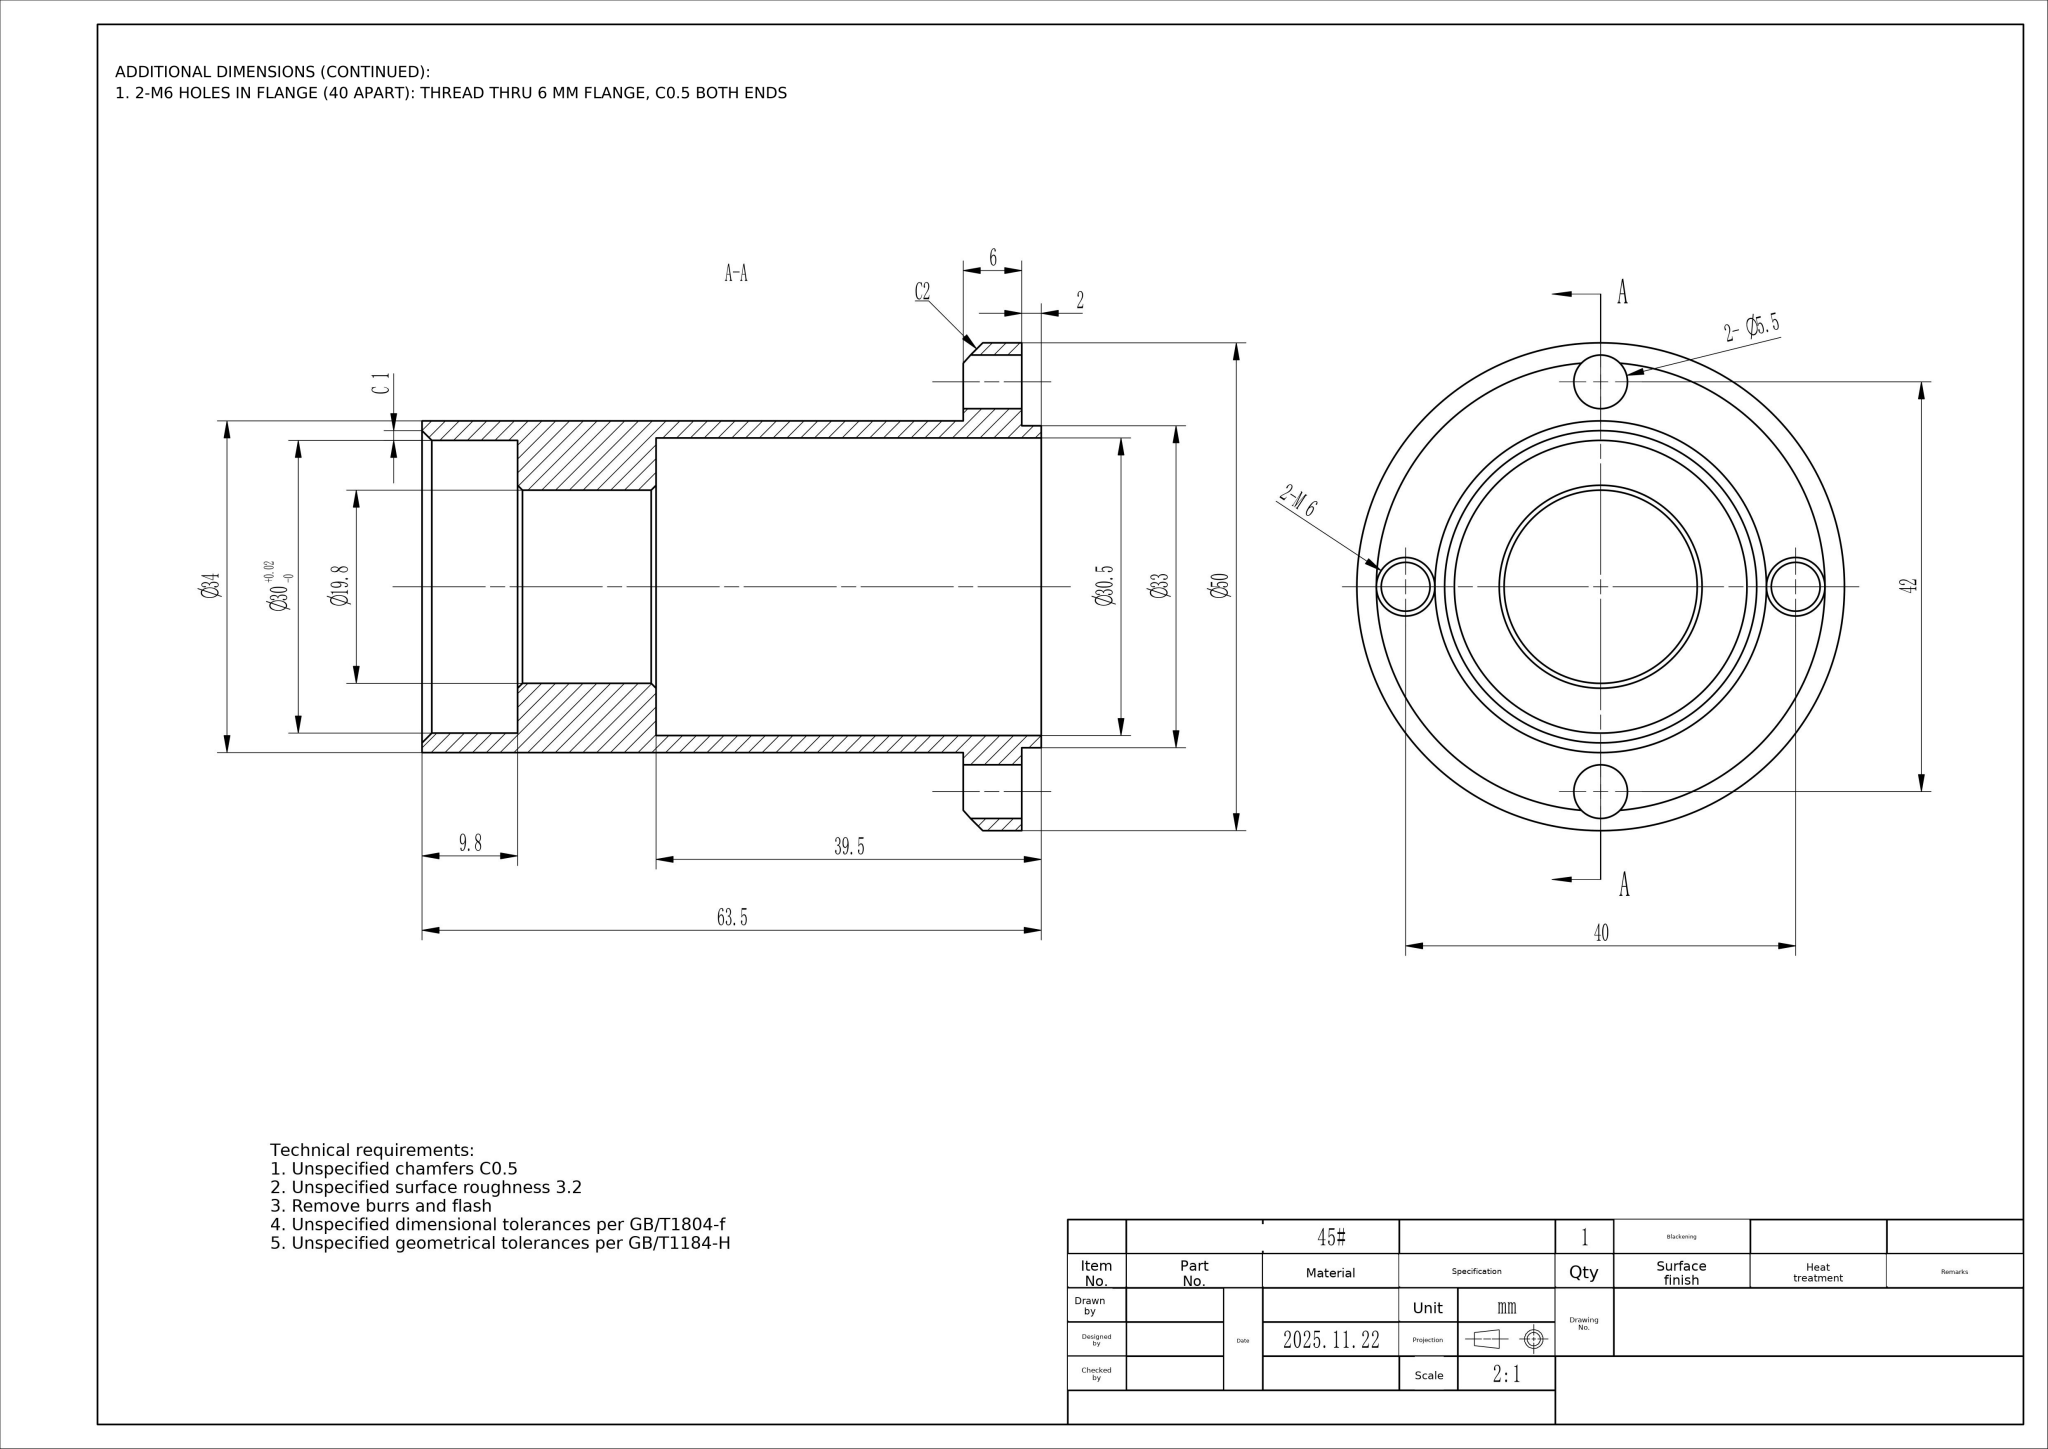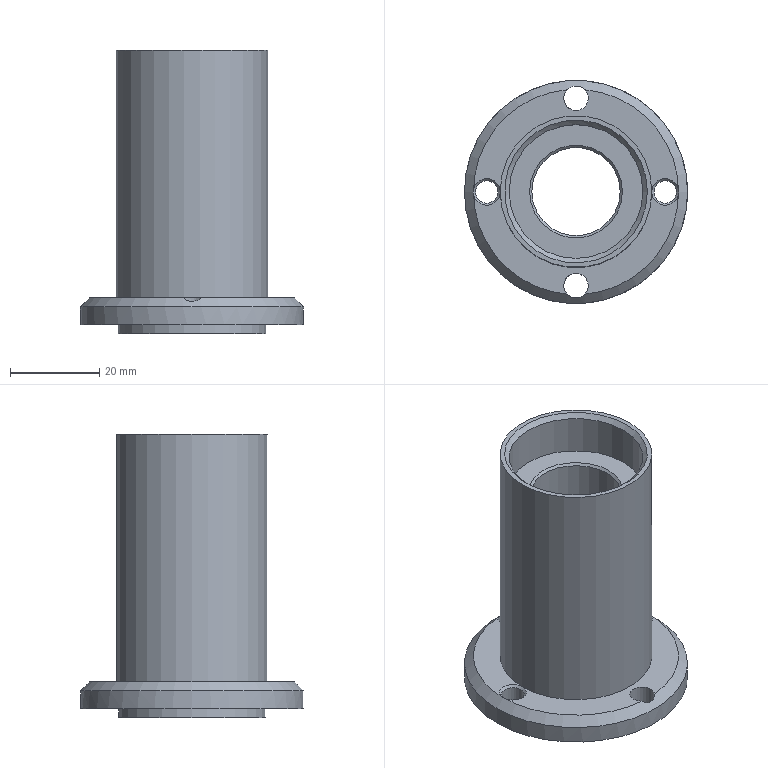Part | NX | mm | 1 solid | 25 faces | box 50 x 50 x 63.5 mm | volume 22825 mm3 | cylinder 10 | cone 8 | plane 7 | commonest cylinder face diameters 5.5 x2 5 x2 19.8 x1 30.5 x1 33 x1 50 x1 34 x1 30 x1
STEP:
#1=CARTESIAN_POINT('',(0.,0.,0.));
#2=DIRECTION('',(0.,0.,1.));
#3=DIRECTION('',(1.,0.,0.));
#4=AXIS2_PLACEMENT_3D('',#1,#2,#3);
#5=(LENGTH_UNIT()NAMED_UNIT(*)SI_UNIT(.MILLI.,.METRE.));
#6=UNCERTAINTY_MEASURE_WITH_UNIT(LENGTH_MEASURE(0.0508),#5,'','');
#7=(NAMED_UNIT(*)PLANE_ANGLE_UNIT()SI_UNIT($,.RADIAN.));
#8=PLANE_ANGLE_MEASURE_WITH_UNIT(PLANE_ANGLE_MEASURE(0.01745),#7);
#9=DIMENSIONAL_EXPONENTS(0.,0.,0.,0.,0.,0.,0.);
#10=(CONVERSION_BASED_UNIT('',#8)NAMED_UNIT(#9)PLANE_ANGLE_UNIT());
#11=(NAMED_UNIT(*)SI_UNIT($,.STERADIAN.)SOLID_ANGLE_UNIT());
#12=(GEOMETRIC_REPRESENTATION_CONTEXT(3)GLOBAL_UNCERTAINTY_ASSIGNED_CONTEXT((#6))GLOBAL_UNIT_ASSIGNED_CONTEXT((#5,#10,#11))REPRESENTATION_CONTEXT('',''));
#13=SHAPE_REPRESENTATION('',(#4),#12);
#14=CARTESIAN_POINT('',(-1.973,22.915,-55.5));
#15=VERTEX_POINT('',#14);
#16=CARTESIAN_POINT('',(1.973,22.915,-55.5));
#17=VERTEX_POINT('',#16);
#18=CARTESIAN_POINT('',(0.,21.,-55.5));
#19=DIRECTION('',(0.,0.,1.));
#20=DIRECTION('',(1.,0.,0.));
#21=AXIS2_PLACEMENT_3D('',#18,#19,#20);
#22=CIRCLE('',#21,2.75);
#23=EDGE_CURVE('',#15,#17,#22,.T.);
#24=ORIENTED_EDGE('',*,*,#23,.F.);
#25=CARTESIAN_POINT('',(-23.,0.,-55.5));
#26=VERTEX_POINT('',#25);
#27=CARTESIAN_POINT('',(0.,0.,-55.5));
#28=DIRECTION('',(0.,0.,1.));
#29=DIRECTION('',(1.,0.,0.));
#30=AXIS2_PLACEMENT_3D('',#27,#28,#29);
#31=CIRCLE('',#30,23.);
#32=EDGE_CURVE('',#15,#26,#31,.T.);
#33=ORIENTED_EDGE('',*,*,#32,.T.);
#34=CARTESIAN_POINT('',(-17.,0.,-55.5));
#35=VERTEX_POINT('',#34);
#36=CARTESIAN_POINT('',(-20.,0.,-55.5));
#37=DIRECTION('',(0.,0.,-1.));
#38=DIRECTION('',(1.,0.,0.));
#39=AXIS2_PLACEMENT_3D('',#36,#37,#38);
#40=CIRCLE('',#39,3.);
#41=EDGE_CURVE('',#26,#35,#40,.T.);
#42=ORIENTED_EDGE('',*,*,#41,.T.);
#43=CARTESIAN_POINT('',(17.,0.,-55.5));
#44=VERTEX_POINT('',#43);
#45=CARTESIAN_POINT('',(0.,0.,-55.5));
#46=DIRECTION('',(0.,0.,1.));
#47=DIRECTION('',(-1.,0.,0.));
#48=AXIS2_PLACEMENT_3D('',#45,#46,#47);
#49=CIRCLE('',#48,17.);
#50=EDGE_CURVE('',#44,#35,#49,.T.);
#51=ORIENTED_EDGE('',*,*,#50,.F.);
#52=CARTESIAN_POINT('',(23.,0.,-55.5));
#53=VERTEX_POINT('',#52);
#54=CARTESIAN_POINT('',(20.,0.,-55.5));
#55=DIRECTION('',(0.,0.,-1.));
#56=DIRECTION('',(1.,0.,0.));
#57=AXIS2_PLACEMENT_3D('',#54,#55,#56);
#58=CIRCLE('',#57,3.);
#59=EDGE_CURVE('',#44,#53,#58,.T.);
#60=ORIENTED_EDGE('',*,*,#59,.T.);
#61=CARTESIAN_POINT('',(0.,0.,-55.5));
#62=DIRECTION('',(0.,0.,1.));
#63=DIRECTION('',(1.,0.,0.));
#64=AXIS2_PLACEMENT_3D('',#61,#62,#63);
#65=CIRCLE('',#64,23.);
#66=EDGE_CURVE('',#53,#17,#65,.T.);
#67=ORIENTED_EDGE('',*,*,#66,.T.);
#68=EDGE_LOOP('',(#24,#33,#42,#51,#60,#67));
#69=FACE_OUTER_BOUND('',#68,.T.);
#70=CARTESIAN_POINT('',(0.,25.,-55.5));
#71=DIRECTION('',(0.,0.,1.));
#72=DIRECTION('',(1.,0.,0.));
#73=AXIS2_PLACEMENT_3D('',#70,#71,#72);
#74=PLANE('',#73);
#75=ADVANCED_FACE('',(#69),#74,.T.);
#76=CARTESIAN_POINT('',(-9.9,0.,-23.5));
#77=VERTEX_POINT('',#76);
#78=CARTESIAN_POINT('',(0.,0.,-23.5));
#79=DIRECTION('',(0.,0.,-1.));
#80=DIRECTION('',(-1.,0.,0.));
#81=AXIS2_PLACEMENT_3D('',#78,#79,#80);
#82=CIRCLE('',#81,9.9);
#83=EDGE_CURVE('',#77,#77,#82,.T.);
#84=ORIENTED_EDGE('',*,*,#83,.T.);
#85=EDGE_LOOP('',(#84));
#86=FACE_BOUND('',#85,.T.);
#87=CARTESIAN_POINT('',(9.9,0.,-10.3));
#88=VERTEX_POINT('',#87);
#89=CARTESIAN_POINT('',(0.,0.,-10.3));
#90=DIRECTION('',(0.,0.,1.));
#91=DIRECTION('',(1.,0.,0.));
#92=AXIS2_PLACEMENT_3D('',#89,#90,#91);
#93=CIRCLE('',#92,9.9);
#94=EDGE_CURVE('',#88,#88,#93,.T.);
#95=ORIENTED_EDGE('',*,*,#94,.T.);
#96=EDGE_LOOP('',(#95));
#97=FACE_BOUND('',#96,.T.);
#98=CARTESIAN_POINT('',(0.,0.,0.));
#99=DIRECTION('',(0.,0.,-1.));
#100=DIRECTION('',(-1.,0.,0.));
#101=AXIS2_PLACEMENT_3D('',#98,#99,#100);
#102=CYLINDRICAL_SURFACE('',#101,9.9);
#103=ADVANCED_FACE('',(#86,#97),#102,.F.);
#104=CARTESIAN_POINT('',(-10.4,0.,-24.));
#105=VERTEX_POINT('',#104);
#106=CARTESIAN_POINT('',(0.,0.,-24.));
#107=DIRECTION('',(0.,0.,1.));
#108=DIRECTION('',(-1.,0.,0.));
#109=AXIS2_PLACEMENT_3D('',#106,#107,#108);
#110=CIRCLE('',#109,10.4);
#111=EDGE_CURVE('',#105,#105,#110,.T.);
#112=ORIENTED_EDGE('',*,*,#111,.T.);
#113=EDGE_LOOP('',(#112));
#114=FACE_BOUND('',#113,.T.);
#115=CARTESIAN_POINT('',(-15.25,0.,-24.));
#116=VERTEX_POINT('',#115);
#117=CARTESIAN_POINT('',(0.,0.,-24.));
#118=DIRECTION('',(0.,0.,1.));
#119=DIRECTION('',(-1.,0.,0.));
#120=AXIS2_PLACEMENT_3D('',#117,#118,#119);
#121=CIRCLE('',#120,15.25);
#122=EDGE_CURVE('',#116,#116,#121,.T.);
#123=ORIENTED_EDGE('',*,*,#122,.F.);
#124=EDGE_LOOP('',(#123));
#125=FACE_BOUND('',#124,.T.);
#126=CARTESIAN_POINT('',(0.,9.9,-24.));
#127=DIRECTION('',(0.,0.,-1.));
#128=DIRECTION('',(-1.,0.,0.));
#129=AXIS2_PLACEMENT_3D('',#126,#127,#128);
#130=PLANE('',#129);
#131=ADVANCED_FACE('',(#114,#125),#130,.T.);
#132=CARTESIAN_POINT('',(-15.25,0.,-63.5));
#133=VERTEX_POINT('',#132);
#134=CARTESIAN_POINT('',(0.,0.,-63.5));
#135=DIRECTION('',(0.,0.,1.));
#136=DIRECTION('',(-1.,0.,0.));
#137=AXIS2_PLACEMENT_3D('',#134,#135,#136);
#138=CIRCLE('',#137,15.25);
#139=EDGE_CURVE('',#133,#133,#138,.T.);
#140=ORIENTED_EDGE('',*,*,#139,.F.);
#141=EDGE_LOOP('',(#140));
#142=FACE_BOUND('',#141,.T.);
#143=ORIENTED_EDGE('',*,*,#122,.T.);
#144=EDGE_LOOP('',(#143));
#145=FACE_BOUND('',#144,.T.);
#146=CARTESIAN_POINT('',(0.,0.,0.));
#147=DIRECTION('',(0.,0.,-1.));
#148=DIRECTION('',(-1.,0.,0.));
#149=AXIS2_PLACEMENT_3D('',#146,#147,#148);
#150=CYLINDRICAL_SURFACE('',#149,15.25);
#151=ADVANCED_FACE('',(#142,#145),#150,.F.);
#152=CARTESIAN_POINT('',(-16.5,0.,-63.5));
#153=VERTEX_POINT('',#152);
#154=CARTESIAN_POINT('',(0.,0.,-63.5));
#155=DIRECTION('',(0.,0.,1.));
#156=DIRECTION('',(-1.,0.,0.));
#157=AXIS2_PLACEMENT_3D('',#154,#155,#156);
#158=CIRCLE('',#157,16.5);
#159=EDGE_CURVE('',#153,#153,#158,.T.);
#160=ORIENTED_EDGE('',*,*,#159,.F.);
#161=EDGE_LOOP('',(#160));
#162=FACE_BOUND('',#161,.T.);
#163=ORIENTED_EDGE('',*,*,#139,.T.);
#164=EDGE_LOOP('',(#163));
#165=FACE_BOUND('',#164,.T.);
#166=CARTESIAN_POINT('',(0.,15.25,-63.5));
#167=DIRECTION('',(0.,0.,-1.));
#168=DIRECTION('',(-1.,0.,0.));
#169=AXIS2_PLACEMENT_3D('',#166,#167,#168);
#170=PLANE('',#169);
#171=ADVANCED_FACE('',(#162,#165),#170,.T.);
#172=CARTESIAN_POINT('',(-16.5,0.,-61.5));
#173=VERTEX_POINT('',#172);
#174=CARTESIAN_POINT('',(0.,0.,-61.5));
#175=DIRECTION('',(0.,0.,1.));
#176=DIRECTION('',(-1.,0.,0.));
#177=AXIS2_PLACEMENT_3D('',#174,#175,#176);
#178=CIRCLE('',#177,16.5);
#179=EDGE_CURVE('',#173,#173,#178,.T.);
#180=ORIENTED_EDGE('',*,*,#179,.F.);
#181=EDGE_LOOP('',(#180));
#182=FACE_BOUND('',#181,.T.);
#183=ORIENTED_EDGE('',*,*,#159,.T.);
#184=EDGE_LOOP('',(#183));
#185=FACE_BOUND('',#184,.T.);
#186=CARTESIAN_POINT('',(0.,0.,0.));
#187=DIRECTION('',(0.,0.,-1.));
#188=DIRECTION('',(-1.,0.,0.));
#189=AXIS2_PLACEMENT_3D('',#186,#187,#188);
#190=CYLINDRICAL_SURFACE('',#189,16.5);
#191=ADVANCED_FACE('',(#182,#185),#190,.T.);
#192=CARTESIAN_POINT('',(17.,0.,-61.5));
#193=VERTEX_POINT('',#192);
#194=CARTESIAN_POINT('',(20.,0.,-61.5));
#195=DIRECTION('',(0.,0.,1.));
#196=DIRECTION('',(-1.,0.,0.));
#197=AXIS2_PLACEMENT_3D('',#194,#195,#196);
#198=CIRCLE('',#197,3.);
#199=EDGE_CURVE('',#193,#193,#198,.T.);
#200=ORIENTED_EDGE('',*,*,#199,.T.);
#201=EDGE_LOOP('',(#200));
#202=FACE_BOUND('',#201,.T.);
#203=CARTESIAN_POINT('',(-23.,0.,-61.5));
#204=VERTEX_POINT('',#203);
#205=CARTESIAN_POINT('',(-20.,0.,-61.5));
#206=DIRECTION('',(0.,0.,1.));
#207=DIRECTION('',(-1.,0.,0.));
#208=AXIS2_PLACEMENT_3D('',#205,#206,#207);
#209=CIRCLE('',#208,3.);
#210=EDGE_CURVE('',#204,#204,#209,.T.);
#211=ORIENTED_EDGE('',*,*,#210,.T.);
#212=EDGE_LOOP('',(#211));
#213=FACE_BOUND('',#212,.T.);
#214=CARTESIAN_POINT('',(-2.75,-21.,-61.5));
#215=VERTEX_POINT('',#214);
#216=CARTESIAN_POINT('',(0.,-21.,-61.5));
#217=DIRECTION('',(0.,0.,-1.));
#218=DIRECTION('',(-1.,0.,0.));
#219=AXIS2_PLACEMENT_3D('',#216,#217,#218);
#220=CIRCLE('',#219,2.75);
#221=EDGE_CURVE('',#215,#215,#220,.T.);
#222=ORIENTED_EDGE('',*,*,#221,.F.);
#223=EDGE_LOOP('',(#222));
#224=FACE_BOUND('',#223,.T.);
#225=CARTESIAN_POINT('',(-2.75,21.,-61.5));
#226=VERTEX_POINT('',#225);
#227=CARTESIAN_POINT('',(0.,21.,-61.5));
#228=DIRECTION('',(0.,0.,-1.));
#229=DIRECTION('',(-1.,0.,0.));
#230=AXIS2_PLACEMENT_3D('',#227,#228,#229);
#231=CIRCLE('',#230,2.75);
#232=EDGE_CURVE('',#226,#226,#231,.T.);
#233=ORIENTED_EDGE('',*,*,#232,.F.);
#234=EDGE_LOOP('',(#233));
#235=FACE_BOUND('',#234,.T.);
#236=CARTESIAN_POINT('',(-25.,0.,-61.5));
#237=VERTEX_POINT('',#236);
#238=CARTESIAN_POINT('',(0.,0.,-61.5));
#239=DIRECTION('',(0.,0.,1.));
#240=DIRECTION('',(-1.,0.,0.));
#241=AXIS2_PLACEMENT_3D('',#238,#239,#240);
#242=CIRCLE('',#241,25.);
#243=EDGE_CURVE('',#237,#237,#242,.T.);
#244=ORIENTED_EDGE('',*,*,#243,.F.);
#245=EDGE_LOOP('',(#244));
#246=FACE_BOUND('',#245,.T.);
#247=ORIENTED_EDGE('',*,*,#179,.T.);
#248=EDGE_LOOP('',(#247));
#249=FACE_BOUND('',#248,.T.);
#250=CARTESIAN_POINT('',(0.,16.5,-61.5));
#251=DIRECTION('',(0.,0.,-1.));
#252=DIRECTION('',(-1.,0.,0.));
#253=AXIS2_PLACEMENT_3D('',#250,#251,#252);
#254=PLANE('',#253);
#255=ADVANCED_FACE('',(#202,#213,#224,#235,#246,#249),#254,.T.);
#256=CARTESIAN_POINT('',(25.,0.,-57.5));
#257=VERTEX_POINT('',#256);
#258=CARTESIAN_POINT('',(0.,0.,-57.5));
#259=DIRECTION('',(0.,0.,-1.));
#260=DIRECTION('',(1.,0.,0.));
#261=AXIS2_PLACEMENT_3D('',#258,#259,#260);
#262=CIRCLE('',#261,25.);
#263=EDGE_CURVE('',#257,#257,#262,.T.);
#264=ORIENTED_EDGE('',*,*,#263,.T.);
#265=EDGE_LOOP('',(#264));
#266=FACE_BOUND('',#265,.T.);
#267=ORIENTED_EDGE('',*,*,#243,.T.);
#268=EDGE_LOOP('',(#267));
#269=FACE_BOUND('',#268,.T.);
#270=CARTESIAN_POINT('',(0.,0.,0.));
#271=DIRECTION('',(0.,0.,-1.));
#272=DIRECTION('',(-1.,0.,0.));
#273=AXIS2_PLACEMENT_3D('',#270,#271,#272);
#274=CYLINDRICAL_SURFACE('',#273,25.);
#275=ADVANCED_FACE('',(#266,#269),#274,.T.);
#276=CARTESIAN_POINT('',(-20.,0.,-55.5));
#277=DIRECTION('',(0.,0.,-1.));
#278=DIRECTION('',(1.,0.,0.));
#279=AXIS2_PLACEMENT_3D('',#276,#277,#278);
#280=CIRCLE('',#279,3.);
#281=EDGE_CURVE('',#35,#26,#280,.T.);
#282=ORIENTED_EDGE('',*,*,#281,.T.);
#283=CARTESIAN_POINT('',(-1.973,-22.915,-55.5));
#284=VERTEX_POINT('',#283);
#285=CARTESIAN_POINT('',(0.,0.,-55.5));
#286=DIRECTION('',(0.,0.,1.));
#287=DIRECTION('',(1.,0.,0.));
#288=AXIS2_PLACEMENT_3D('',#285,#286,#287);
#289=CIRCLE('',#288,23.);
#290=EDGE_CURVE('',#26,#284,#289,.T.);
#291=ORIENTED_EDGE('',*,*,#290,.T.);
#292=CARTESIAN_POINT('',(1.973,-22.915,-55.5));
#293=VERTEX_POINT('',#292);
#294=CARTESIAN_POINT('',(0.,-21.,-55.5));
#295=DIRECTION('',(0.,0.,1.));
#296=DIRECTION('',(1.,0.,0.));
#297=AXIS2_PLACEMENT_3D('',#294,#295,#296);
#298=CIRCLE('',#297,2.75);
#299=EDGE_CURVE('',#293,#284,#298,.T.);
#300=ORIENTED_EDGE('',*,*,#299,.F.);
#301=CARTESIAN_POINT('',(0.,0.,-55.5));
#302=DIRECTION('',(0.,0.,1.));
#303=DIRECTION('',(1.,0.,0.));
#304=AXIS2_PLACEMENT_3D('',#301,#302,#303);
#305=CIRCLE('',#304,23.);
#306=EDGE_CURVE('',#293,#53,#305,.T.);
#307=ORIENTED_EDGE('',*,*,#306,.T.);
#308=CARTESIAN_POINT('',(20.,0.,-55.5));
#309=DIRECTION('',(0.,0.,-1.));
#310=DIRECTION('',(1.,0.,0.));
#311=AXIS2_PLACEMENT_3D('',#308,#309,#310);
#312=CIRCLE('',#311,3.);
#313=EDGE_CURVE('',#53,#44,#312,.T.);
#314=ORIENTED_EDGE('',*,*,#313,.T.);
#315=CARTESIAN_POINT('',(0.,0.,-55.5));
#316=DIRECTION('',(0.,0.,1.));
#317=DIRECTION('',(-1.,0.,0.));
#318=AXIS2_PLACEMENT_3D('',#315,#316,#317);
#319=CIRCLE('',#318,17.);
#320=EDGE_CURVE('',#35,#44,#319,.T.);
#321=ORIENTED_EDGE('',*,*,#320,.F.);
#322=EDGE_LOOP('',(#282,#291,#300,#307,#314,#321));
#323=FACE_OUTER_BOUND('',#322,.T.);
#324=CARTESIAN_POINT('',(0.,25.,-55.5));
#325=DIRECTION('',(0.,0.,1.));
#326=DIRECTION('',(1.,0.,0.));
#327=AXIS2_PLACEMENT_3D('',#324,#325,#326);
#328=PLANE('',#327);
#329=ADVANCED_FACE('',(#323),#328,.T.);
#330=CARTESIAN_POINT('',(-17.,0.,0.));
#331=VERTEX_POINT('',#330);
#332=CARTESIAN_POINT('',(0.,0.,0.));
#333=DIRECTION('',(0.,0.,1.));
#334=DIRECTION('',(-1.,0.,0.));
#335=AXIS2_PLACEMENT_3D('',#332,#333,#334);
#336=CIRCLE('',#335,17.);
#337=EDGE_CURVE('',#331,#331,#336,.T.);
#338=ORIENTED_EDGE('',*,*,#337,.F.);
#339=EDGE_LOOP('',(#338));
#340=FACE_BOUND('',#339,.T.);
#341=ORIENTED_EDGE('',*,*,#320,.T.);
#342=ORIENTED_EDGE('',*,*,#50,.T.);
#343=EDGE_LOOP('',(#341,#342));
#344=FACE_BOUND('',#343,.T.);
#345=CARTESIAN_POINT('',(0.,0.,0.));
#346=DIRECTION('',(0.,0.,-1.));
#347=DIRECTION('',(-1.,0.,0.));
#348=AXIS2_PLACEMENT_3D('',#345,#346,#347);
#349=CYLINDRICAL_SURFACE('',#348,17.);
#350=ADVANCED_FACE('',(#340,#344),#349,.T.);
#351=CARTESIAN_POINT('',(16.,0.,0.));
#352=VERTEX_POINT('',#351);
#353=CARTESIAN_POINT('',(0.,0.,0.));
#354=DIRECTION('',(0.,0.,-1.));
#355=DIRECTION('',(1.,0.,0.));
#356=AXIS2_PLACEMENT_3D('',#353,#354,#355);
#357=CIRCLE('',#356,16.);
#358=EDGE_CURVE('',#352,#352,#357,.T.);
#359=ORIENTED_EDGE('',*,*,#358,.T.);
#360=EDGE_LOOP('',(#359));
#361=FACE_BOUND('',#360,.T.);
#362=ORIENTED_EDGE('',*,*,#337,.T.);
#363=EDGE_LOOP('',(#362));
#364=FACE_BOUND('',#363,.T.);
#365=CARTESIAN_POINT('',(0.,17.,0.));
#366=DIRECTION('',(0.,0.,1.));
#367=DIRECTION('',(1.,0.,0.));
#368=AXIS2_PLACEMENT_3D('',#365,#366,#367);
#369=PLANE('',#368);
#370=ADVANCED_FACE('',(#361,#364),#369,.T.);
#371=CARTESIAN_POINT('',(15.,0.,-1.));
#372=VERTEX_POINT('',#371);
#373=CARTESIAN_POINT('',(0.,0.,-1.));
#374=DIRECTION('',(0.,0.,1.));
#375=DIRECTION('',(1.,0.,0.));
#376=AXIS2_PLACEMENT_3D('',#373,#374,#375);
#377=CIRCLE('',#376,15.);
#378=EDGE_CURVE('',#372,#372,#377,.T.);
#379=ORIENTED_EDGE('',*,*,#378,.T.);
#380=EDGE_LOOP('',(#379));
#381=FACE_BOUND('',#380,.T.);
#382=CARTESIAN_POINT('',(-15.,0.,-9.8));
#383=VERTEX_POINT('',#382);
#384=CARTESIAN_POINT('',(0.,0.,-9.8));
#385=DIRECTION('',(0.,0.,1.));
#386=DIRECTION('',(-1.,0.,0.));
#387=AXIS2_PLACEMENT_3D('',#384,#385,#386);
#388=CIRCLE('',#387,15.);
#389=EDGE_CURVE('',#383,#383,#388,.T.);
#390=ORIENTED_EDGE('',*,*,#389,.F.);
#391=EDGE_LOOP('',(#390));
#392=FACE_BOUND('',#391,.T.);
#393=CARTESIAN_POINT('',(0.,0.,0.));
#394=DIRECTION('',(0.,0.,-1.));
#395=DIRECTION('',(-1.,0.,0.));
#396=AXIS2_PLACEMENT_3D('',#393,#394,#395);
#397=CYLINDRICAL_SURFACE('',#396,15.);
#398=ADVANCED_FACE('',(#381,#392),#397,.F.);
#399=CARTESIAN_POINT('',(10.4,0.,-9.8));
#400=VERTEX_POINT('',#399);
#401=CARTESIAN_POINT('',(0.,0.,-9.8));
#402=DIRECTION('',(0.,0.,-1.));
#403=DIRECTION('',(1.,0.,0.));
#404=AXIS2_PLACEMENT_3D('',#401,#402,#403);
#405=CIRCLE('',#404,10.4);
#406=EDGE_CURVE('',#400,#400,#405,.T.);
#407=ORIENTED_EDGE('',*,*,#406,.T.);
#408=EDGE_LOOP('',(#407));
#409=FACE_BOUND('',#408,.T.);
#410=ORIENTED_EDGE('',*,*,#389,.T.);
#411=EDGE_LOOP('',(#410));
#412=FACE_BOUND('',#411,.T.);
#413=CARTESIAN_POINT('',(0.,15.,-9.8));
#414=DIRECTION('',(0.,0.,1.));
#415=DIRECTION('',(1.,0.,0.));
#416=AXIS2_PLACEMENT_3D('',#413,#414,#415);
#417=PLANE('',#416);
#418=ADVANCED_FACE('',(#409,#412),#417,.T.);
#419=ORIENTED_EDGE('',*,*,#232,.T.);
#420=EDGE_LOOP('',(#419));
#421=FACE_BOUND('',#420,.T.);
#422=ORIENTED_EDGE('',*,*,#23,.T.);
#423=CARTESIAN_POINT('',(1.973,22.915,-55.5));
#424=CARTESIAN_POINT('',(1.792,23.102,-55.67));
#425=CARTESIAN_POINT('',(1.573,23.274,-55.825));
#426=CARTESIAN_POINT('',(1.323,23.411,-55.948));
#427=CARTESIAN_POINT('',(1.113,23.526,-56.051));
#428=CARTESIAN_POINT('',(0.8756,23.619,-56.134));
#429=CARTESIAN_POINT('',(0.6267,23.678,-56.186));
#430=CARTESIAN_POINT('',(0.3767,23.736,-56.238));
#431=CARTESIAN_POINT('',(0.1073,23.76,-56.259));
#432=CARTESIAN_POINT('',(-0.154,23.746,-56.246));
#433=CARTESIAN_POINT('',(-0.3876,23.733,-56.235));
#434=CARTESIAN_POINT('',(-0.6208,23.689,-56.196));
#435=CARTESIAN_POINT('',(-0.8362,23.62,-56.135));
#436=CARTESIAN_POINT('',(-1.056,23.55,-56.072));
#437=CARTESIAN_POINT('',(-1.263,23.452,-55.985));
#438=CARTESIAN_POINT('',(-1.447,23.338,-55.883));
#439=CARTESIAN_POINT('',(-1.646,23.215,-55.773));
#440=CARTESIAN_POINT('',(-1.823,23.071,-55.642));
#441=CARTESIAN_POINT('',(-1.973,22.915,-55.5));
#442=B_SPLINE_CURVE_WITH_KNOTS('',3,(#423,#424,#425,#426,#427,#428,#429,#430,#431,#432,#433,#434,#435,#436,#437,#438,#439,#440,#441),.UNSPECIFIED.,.F.,.F.,(4,3,3,3,3,3,4),(0.,0.1988,0.3655,0.5334,0.6828,0.8353,1.),.UNSPECIFIED.);
#443=EDGE_CURVE('',#17,#15,#442,.T.);
#444=ORIENTED_EDGE('',*,*,#443,.T.);
#445=EDGE_LOOP('',(#422,#444));
#446=FACE_BOUND('',#445,.T.);
#447=CARTESIAN_POINT('',(0.,21.,-97.));
#448=DIRECTION('',(0.,0.,1.));
#449=DIRECTION('',(1.,0.,0.));
#450=AXIS2_PLACEMENT_3D('',#447,#448,#449);
#451=CYLINDRICAL_SURFACE('',#450,2.75);
#452=ADVANCED_FACE('',(#421,#446),#451,.F.);
#453=ORIENTED_EDGE('',*,*,#221,.T.);
#454=EDGE_LOOP('',(#453));
#455=FACE_BOUND('',#454,.T.);
#456=ORIENTED_EDGE('',*,*,#299,.T.);
#457=CARTESIAN_POINT('',(-1.973,-22.915,-55.5));
#458=CARTESIAN_POINT('',(-1.792,-23.102,-55.67));
#459=CARTESIAN_POINT('',(-1.573,-23.274,-55.825));
#460=CARTESIAN_POINT('',(-1.323,-23.411,-55.948));
#461=CARTESIAN_POINT('',(-1.113,-23.526,-56.051));
#462=CARTESIAN_POINT('',(-0.8756,-23.619,-56.134));
#463=CARTESIAN_POINT('',(-0.6267,-23.678,-56.186));
#464=CARTESIAN_POINT('',(-0.3767,-23.736,-56.238));
#465=CARTESIAN_POINT('',(-0.1073,-23.76,-56.259));
#466=CARTESIAN_POINT('',(0.154,-23.746,-56.246));
#467=CARTESIAN_POINT('',(0.3876,-23.733,-56.235));
#468=CARTESIAN_POINT('',(0.6208,-23.689,-56.196));
#469=CARTESIAN_POINT('',(0.8362,-23.62,-56.135));
#470=CARTESIAN_POINT('',(1.056,-23.55,-56.072));
#471=CARTESIAN_POINT('',(1.263,-23.452,-55.985));
#472=CARTESIAN_POINT('',(1.447,-23.338,-55.883));
#473=CARTESIAN_POINT('',(1.646,-23.215,-55.773));
#474=CARTESIAN_POINT('',(1.823,-23.071,-55.642));
#475=CARTESIAN_POINT('',(1.973,-22.915,-55.5));
#476=B_SPLINE_CURVE_WITH_KNOTS('',3,(#457,#458,#459,#460,#461,#462,#463,#464,#465,#466,#467,#468,#469,#470,#471,#472,#473,#474,#475),.UNSPECIFIED.,.F.,.F.,(4,3,3,3,3,3,4),(0.,0.1988,0.3655,0.5334,0.6828,0.8353,1.),.UNSPECIFIED.);
#477=EDGE_CURVE('',#284,#293,#476,.T.);
#478=ORIENTED_EDGE('',*,*,#477,.T.);
#479=EDGE_LOOP('',(#456,#478));
#480=FACE_BOUND('',#479,.T.);
#481=CARTESIAN_POINT('',(0.,-21.,-97.));
#482=DIRECTION('',(0.,0.,1.));
#483=DIRECTION('',(1.,0.,0.));
#484=AXIS2_PLACEMENT_3D('',#481,#482,#483);
#485=CYLINDRICAL_SURFACE('',#484,2.75);
#486=ADVANCED_FACE('',(#455,#480),#485,.F.);
#487=CARTESIAN_POINT('',(-17.5,0.,-56.));
#488=VERTEX_POINT('',#487);
#489=CARTESIAN_POINT('',(-20.,0.,-56.));
#490=DIRECTION('',(0.,0.,1.));
#491=DIRECTION('',(1.,0.,0.));
#492=AXIS2_PLACEMENT_3D('',#489,#490,#491);
#493=CIRCLE('',#492,2.5);
#494=EDGE_CURVE('',#488,#488,#493,.T.);
#495=ORIENTED_EDGE('',*,*,#494,.T.);
#496=EDGE_LOOP('',(#495));
#497=FACE_BOUND('',#496,.T.);
#498=CARTESIAN_POINT('',(-22.5,0.,-61.));
#499=VERTEX_POINT('',#498);
#500=CARTESIAN_POINT('',(-20.,0.,-61.));
#501=DIRECTION('',(0.,0.,-1.));
#502=DIRECTION('',(-1.,0.,0.));
#503=AXIS2_PLACEMENT_3D('',#500,#501,#502);
#504=CIRCLE('',#503,2.5);
#505=EDGE_CURVE('',#499,#499,#504,.T.);
#506=ORIENTED_EDGE('',*,*,#505,.T.);
#507=EDGE_LOOP('',(#506));
#508=FACE_BOUND('',#507,.T.);
#509=CARTESIAN_POINT('',(-20.,0.,-61.5));
#510=DIRECTION('',(0.,0.,1.));
#511=DIRECTION('',(1.,0.,0.));
#512=AXIS2_PLACEMENT_3D('',#509,#510,#511);
#513=CYLINDRICAL_SURFACE('',#512,2.5);
#514=ADVANCED_FACE('',(#497,#508),#513,.F.);
#515=ORIENTED_EDGE('',*,*,#505,.F.);
#516=EDGE_LOOP('',(#515));
#517=FACE_BOUND('',#516,.T.);
#518=ORIENTED_EDGE('',*,*,#210,.F.);
#519=EDGE_LOOP('',(#518));
#520=FACE_BOUND('',#519,.T.);
#521=CARTESIAN_POINT('',(-20.,0.,-61.5));
#522=DIRECTION('',(0.,0.,-1.));
#523=DIRECTION('',(-1.,0.,-0.));
#524=AXIS2_PLACEMENT_3D('',#521,#522,#523);
#525=CONICAL_SURFACE('',#524,3.,45.);
#526=ADVANCED_FACE('',(#517,#520),#525,.F.);
#527=ORIENTED_EDGE('',*,*,#281,.F.);
#528=ORIENTED_EDGE('',*,*,#41,.F.);
#529=EDGE_LOOP('',(#527,#528));
#530=FACE_BOUND('',#529,.T.);
#531=ORIENTED_EDGE('',*,*,#494,.F.);
#532=EDGE_LOOP('',(#531));
#533=FACE_BOUND('',#532,.T.);
#534=CARTESIAN_POINT('',(-20.,0.,-56.));
#535=DIRECTION('',(0.,0.,1.));
#536=DIRECTION('',(1.,0.,-0.));
#537=AXIS2_PLACEMENT_3D('',#534,#535,#536);
#538=CONICAL_SURFACE('',#537,2.5,45.);
#539=ADVANCED_FACE('',(#530,#533),#538,.F.);
#540=CARTESIAN_POINT('',(22.5,0.,-56.));
#541=VERTEX_POINT('',#540);
#542=CARTESIAN_POINT('',(20.,0.,-56.));
#543=DIRECTION('',(0.,0.,1.));
#544=DIRECTION('',(1.,0.,0.));
#545=AXIS2_PLACEMENT_3D('',#542,#543,#544);
#546=CIRCLE('',#545,2.5);
#547=EDGE_CURVE('',#541,#541,#546,.T.);
#548=ORIENTED_EDGE('',*,*,#547,.T.);
#549=EDGE_LOOP('',(#548));
#550=FACE_BOUND('',#549,.T.);
#551=CARTESIAN_POINT('',(17.5,0.,-61.));
#552=VERTEX_POINT('',#551);
#553=CARTESIAN_POINT('',(20.,0.,-61.));
#554=DIRECTION('',(0.,0.,-1.));
#555=DIRECTION('',(-1.,0.,0.));
#556=AXIS2_PLACEMENT_3D('',#553,#554,#555);
#557=CIRCLE('',#556,2.5);
#558=EDGE_CURVE('',#552,#552,#557,.T.);
#559=ORIENTED_EDGE('',*,*,#558,.T.);
#560=EDGE_LOOP('',(#559));
#561=FACE_BOUND('',#560,.T.);
#562=CARTESIAN_POINT('',(20.,0.,-61.5));
#563=DIRECTION('',(0.,0.,1.));
#564=DIRECTION('',(1.,0.,0.));
#565=AXIS2_PLACEMENT_3D('',#562,#563,#564);
#566=CYLINDRICAL_SURFACE('',#565,2.5);
#567=ADVANCED_FACE('',(#550,#561),#566,.F.);
#568=ORIENTED_EDGE('',*,*,#558,.F.);
#569=EDGE_LOOP('',(#568));
#570=FACE_BOUND('',#569,.T.);
#571=ORIENTED_EDGE('',*,*,#199,.F.);
#572=EDGE_LOOP('',(#571));
#573=FACE_BOUND('',#572,.T.);
#574=CARTESIAN_POINT('',(20.,0.,-61.5));
#575=DIRECTION('',(0.,0.,-1.));
#576=DIRECTION('',(-1.,0.,-0.));
#577=AXIS2_PLACEMENT_3D('',#574,#575,#576);
#578=CONICAL_SURFACE('',#577,3.,45.);
#579=ADVANCED_FACE('',(#570,#573),#578,.F.);
#580=ORIENTED_EDGE('',*,*,#59,.F.);
#581=ORIENTED_EDGE('',*,*,#313,.F.);
#582=EDGE_LOOP('',(#580,#581));
#583=FACE_BOUND('',#582,.T.);
#584=ORIENTED_EDGE('',*,*,#547,.F.);
#585=EDGE_LOOP('',(#584));
#586=FACE_BOUND('',#585,.T.);
#587=CARTESIAN_POINT('',(20.,0.,-56.));
#588=DIRECTION('',(0.,0.,1.));
#589=DIRECTION('',(1.,0.,-0.));
#590=AXIS2_PLACEMENT_3D('',#587,#588,#589);
#591=CONICAL_SURFACE('',#590,2.5,45.);
#592=ADVANCED_FACE('',(#583,#586),#591,.F.);
#593=ORIENTED_EDGE('',*,*,#83,.F.);
#594=EDGE_LOOP('',(#593));
#595=FACE_BOUND('',#594,.T.);
#596=ORIENTED_EDGE('',*,*,#111,.F.);
#597=EDGE_LOOP('',(#596));
#598=FACE_BOUND('',#597,.T.);
#599=CARTESIAN_POINT('',(0.,0.,-24.));
#600=DIRECTION('',(0.,0.,-1.));
#601=DIRECTION('',(-1.,0.,-0.));
#602=AXIS2_PLACEMENT_3D('',#599,#600,#601);
#603=CONICAL_SURFACE('',#602,10.4,45.);
#604=ADVANCED_FACE('',(#595,#598),#603,.F.);
#605=ORIENTED_EDGE('',*,*,#406,.F.);
#606=EDGE_LOOP('',(#605));
#607=FACE_BOUND('',#606,.T.);
#608=ORIENTED_EDGE('',*,*,#94,.F.);
#609=EDGE_LOOP('',(#608));
#610=FACE_BOUND('',#609,.T.);
#611=CARTESIAN_POINT('',(0.,0.,-10.3));
#612=DIRECTION('',(0.,0.,1.));
#613=DIRECTION('',(1.,0.,0.));
#614=AXIS2_PLACEMENT_3D('',#611,#612,#613);
#615=CONICAL_SURFACE('',#614,9.9,45.);
#616=ADVANCED_FACE('',(#607,#610),#615,.F.);
#617=ORIENTED_EDGE('',*,*,#263,.F.);
#618=EDGE_LOOP('',(#617));
#619=FACE_BOUND('',#618,.T.);
#620=ORIENTED_EDGE('',*,*,#290,.F.);
#621=ORIENTED_EDGE('',*,*,#32,.F.);
#622=ORIENTED_EDGE('',*,*,#443,.F.);
#623=ORIENTED_EDGE('',*,*,#66,.F.);
#624=ORIENTED_EDGE('',*,*,#306,.F.);
#625=ORIENTED_EDGE('',*,*,#477,.F.);
#626=EDGE_LOOP('',(#620,#621,#622,#623,#624,#625));
#627=FACE_BOUND('',#626,.T.);
#628=CARTESIAN_POINT('',(0.,0.,-55.5));
#629=DIRECTION('',(0.,0.,-1.));
#630=DIRECTION('',(-1.,0.,-0.));
#631=AXIS2_PLACEMENT_3D('',#628,#629,#630);
#632=CONICAL_SURFACE('',#631,23.,45.);
#633=ADVANCED_FACE('',(#619,#627),#632,.T.);
#634=ORIENTED_EDGE('',*,*,#358,.F.);
#635=EDGE_LOOP('',(#634));
#636=FACE_BOUND('',#635,.T.);
#637=ORIENTED_EDGE('',*,*,#378,.F.);
#638=EDGE_LOOP('',(#637));
#639=FACE_BOUND('',#638,.T.);
#640=CARTESIAN_POINT('',(0.,0.,-1.));
#641=DIRECTION('',(0.,0.,1.));
#642=DIRECTION('',(1.,0.,-0.));
#643=AXIS2_PLACEMENT_3D('',#640,#641,#642);
#644=CONICAL_SURFACE('',#643,15.,45.);
#645=ADVANCED_FACE('',(#636,#639),#644,.F.);
#646=CLOSED_SHELL('',(#75,#103,#131,#151,#171,#191,#255,#275,#329,#350,#370,#398,#418,#452,#486,#514,#526,#539,#567,#579,#592,#604,#616,#633,#645));
#647=MANIFOLD_SOLID_BREP('',#646);
#648=ADVANCED_BREP_SHAPE_REPRESENTATION('',(#647),#12);
#649=SHAPE_REPRESENTATION_RELATIONSHIP('','',#13,#648);
#650=PRESENTATION_LAYER_ASSIGNMENT('','',(#647));
#651=COLOUR_RGB('',0.5961,0.6667,0.6863);
#652=FILL_AREA_STYLE_COLOUR('',#651);
#653=FILL_AREA_STYLE('',(#652));
#654=SURFACE_STYLE_FILL_AREA(#653);
#655=SURFACE_SIDE_STYLE('',(#654));
#656=SURFACE_STYLE_USAGE(.BOTH.,#655);
#657=PRESENTATION_STYLE_ASSIGNMENT((#656));
#658=STYLED_ITEM('',(#657),#647);
#659=MECHANICAL_DESIGN_GEOMETRIC_PRESENTATION_REPRESENTATION('',(#658),#12);